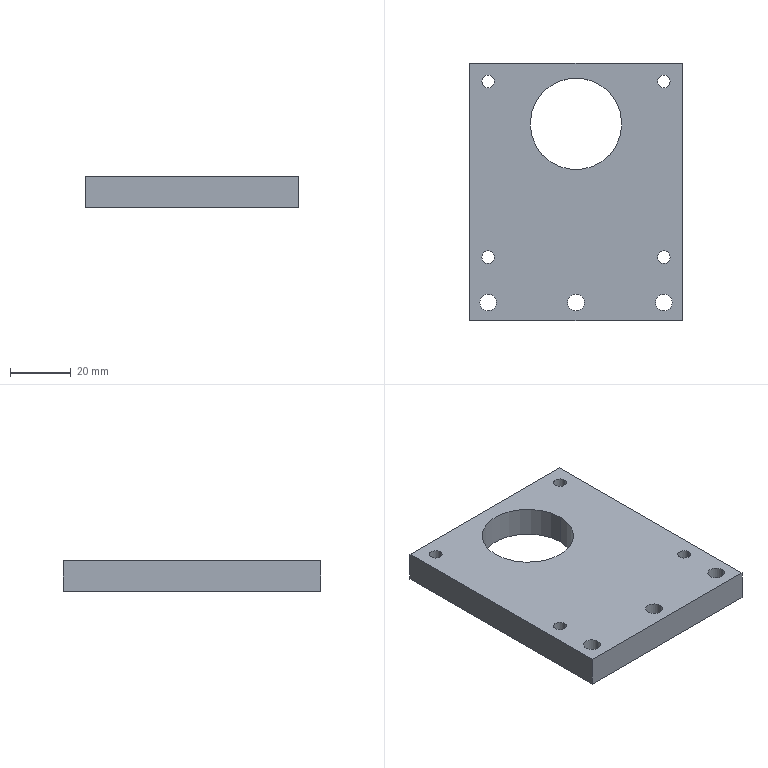Component | SolidWorks | LD101-02--Q1000-Q16-1.SLDQ1SM-1_LD101-02--Q1108-1-1 | 1 solid | 31 faces | box 70 x 85 x 10 mm | volume 50388 mm3 | cylinder 22 | plane 9 | commonest cylinder face diameters 4.2 x8 9 x6 5.5 x6 30.2 x2 | material AL6061
build123d program:
from build123d import *

# Parameters (mm, degrees)
SKETCH1_W                                          = 70
SKETCH1_H                                          = 85
SKETCH1_R                                          = 15.1
BOSS_EXTRUDE1_DEPTH                                = 5
HOLE_SIZE_FOR_HEX_SOCKET_HEAD_CAP_SCRE_D           = 5.5
HOLE_SIZE_FOR_HEX_SOCKET_HEAD_CAP_SCRE_CBORE_D     = 9
HOLE_SIZE_FOR_HEX_SOCKET_HEAD_CAP_SCRE_CBORE_DEPTH = 5.7
M5_TAPPED_HOLE1_D                                  = 4.2


with BuildPart() as part:
    # Sketch1 → Boss-Extrude1 (new, symmetric)
    with BuildSketch(Plane.XY):
        Rectangle(SKETCH1_W, SKETCH1_H)
        with Locations((0, 22.5)):
            Circle(SKETCH1_R, mode=Mode.SUBTRACT)
    extrude(amount=BOSS_EXTRUDE1_DEPTH, both=True)

    # Hole Size _for_ Hex Socket Head Cap Scre (through all)
    with Locations(Plane.XY.offset(5)):
        with Locations((-29, -36.5), (0, -36.5), (29, -36.5)):
            CounterBoreHole(HOLE_SIZE_FOR_HEX_SOCKET_HEAD_CAP_SCRE_D / 2, HOLE_SIZE_FOR_HEX_SOCKET_HEAD_CAP_SCRE_CBORE_D / 2, HOLE_SIZE_FOR_HEX_SOCKET_HEAD_CAP_SCRE_CBORE_DEPTH)

    # M5 Tapped Hole1 (through all)
    with Locations(Plane(origin=(0, 0, -5), x_dir=(-1, 0, 0), z_dir=(0, 0, -1))):
        with Locations((-28.991, -21.491), (28.991, -21.491), (-28.991, 36.491), (28.991, 36.491)):
            Hole(M5_TAPPED_HOLE1_D / 2)


solid = part.part

# Placed as in the assembly
solid = solid.moved(Location((-753.29, -98.397, -75.743), (-180, 0, 180)))
STEP:
#1=CARTESIAN_POINT('',(-30.881,-4.72,-3.179));
#2=VERTEX_POINT('',#1);
#3=CARTESIAN_POINT('',(-30.716,-4.72,-3.179));
#4=VERTEX_POINT('',#3);
#5=CARTESIAN_POINT('',(-30.798,-4.72,-3.179));
#6=DIRECTION('',(-0.,-0.,1.));
#7=DIRECTION('',(1.,0.,0.));
#8=AXIS2_PLACEMENT_3D('',#5,#6,#7);
#9=CIRCLE('',#8,0.08268);
#10=EDGE_CURVE('',#2,#4,#9,.T.);
#11=ORIENTED_EDGE('',*,*,#10,.F.);
#12=CARTESIAN_POINT('',(-30.881,-4.72,-2.785));
#13=VERTEX_POINT('',#12);
#14=CARTESIAN_POINT('',(-30.881,-4.72,-2.785));
#15=DIRECTION('',(-0.,-0.,1.));
#16=VECTOR('',#15,39.37);
#17=LINE('',#14,#16);
#18=EDGE_CURVE('',#2,#13,#17,.T.);
#19=ORIENTED_EDGE('',*,*,#18,.T.);
#20=CARTESIAN_POINT('',(-30.716,-4.72,-2.785));
#21=VERTEX_POINT('',#20);
#22=CARTESIAN_POINT('',(-30.798,-4.72,-2.785));
#23=DIRECTION('',(-0.,-0.,1.));
#24=DIRECTION('',(1.,0.,0.));
#25=AXIS2_PLACEMENT_3D('',#22,#23,#24);
#26=CIRCLE('',#25,0.08268);
#27=EDGE_CURVE('',#13,#21,#26,.T.);
#28=ORIENTED_EDGE('',*,*,#27,.T.);
#29=CARTESIAN_POINT('',(-30.716,-4.72,-2.785));
#30=DIRECTION('',(-0.,-0.,1.));
#31=VECTOR('',#30,39.37);
#32=LINE('',#29,#31);
#33=EDGE_CURVE('',#4,#21,#32,.T.);
#34=ORIENTED_EDGE('',*,*,#33,.F.);
#35=EDGE_LOOP('',(#11,#19,#28,#34));
#36=FACE_OUTER_BOUND('',#35,.T.);
#37=CARTESIAN_POINT('',(-30.798,-4.72,-2.785));
#38=DIRECTION('',(-0.,-0.,1.));
#39=DIRECTION('',(1.,0.,0.));
#40=AXIS2_PLACEMENT_3D('',#37,#38,#39);
#41=CYLINDRICAL_SURFACE('',#40,0.08268);
#42=ADVANCED_FACE('',(#36),#41,.F.);
#43=CARTESIAN_POINT('',(-28.598,-4.72,-3.179));
#44=VERTEX_POINT('',#43);
#45=CARTESIAN_POINT('',(-28.433,-4.72,-3.179));
#46=VERTEX_POINT('',#45);
#47=CARTESIAN_POINT('',(-28.516,-4.72,-3.179));
#48=DIRECTION('',(-0.,-0.,1.));
#49=DIRECTION('',(1.,0.,0.));
#50=AXIS2_PLACEMENT_3D('',#47,#48,#49);
#51=CIRCLE('',#50,0.08268);
#52=EDGE_CURVE('',#44,#46,#51,.T.);
#53=ORIENTED_EDGE('',*,*,#52,.F.);
#54=CARTESIAN_POINT('',(-28.598,-4.72,-2.785));
#55=VERTEX_POINT('',#54);
#56=CARTESIAN_POINT('',(-28.598,-4.72,-2.785));
#57=DIRECTION('',(-0.,-0.,1.));
#58=VECTOR('',#57,39.37);
#59=LINE('',#56,#58);
#60=EDGE_CURVE('',#44,#55,#59,.T.);
#61=ORIENTED_EDGE('',*,*,#60,.T.);
#62=CARTESIAN_POINT('',(-28.433,-4.72,-2.785));
#63=VERTEX_POINT('',#62);
#64=CARTESIAN_POINT('',(-28.516,-4.72,-2.785));
#65=DIRECTION('',(-0.,-0.,1.));
#66=DIRECTION('',(1.,0.,0.));
#67=AXIS2_PLACEMENT_3D('',#64,#65,#66);
#68=CIRCLE('',#67,0.08268);
#69=EDGE_CURVE('',#55,#63,#68,.T.);
#70=ORIENTED_EDGE('',*,*,#69,.T.);
#71=CARTESIAN_POINT('',(-28.433,-4.72,-2.785));
#72=DIRECTION('',(-0.,-0.,1.));
#73=VECTOR('',#72,39.37);
#74=LINE('',#71,#73);
#75=EDGE_CURVE('',#46,#63,#74,.T.);
#76=ORIENTED_EDGE('',*,*,#75,.F.);
#77=EDGE_LOOP('',(#53,#61,#70,#76));
#78=FACE_OUTER_BOUND('',#77,.T.);
#79=CARTESIAN_POINT('',(-28.516,-4.72,-2.785));
#80=DIRECTION('',(-0.,-0.,1.));
#81=DIRECTION('',(1.,0.,0.));
#82=AXIS2_PLACEMENT_3D('',#79,#80,#81);
#83=CYLINDRICAL_SURFACE('',#82,0.08268);
#84=ADVANCED_FACE('',(#78),#83,.F.);
#85=CARTESIAN_POINT('',(-30.881,-2.437,-3.179));
#86=VERTEX_POINT('',#85);
#87=CARTESIAN_POINT('',(-30.716,-2.437,-3.179));
#88=VERTEX_POINT('',#87);
#89=CARTESIAN_POINT('',(-30.798,-2.437,-3.179));
#90=DIRECTION('',(-0.,-0.,1.));
#91=DIRECTION('',(1.,0.,0.));
#92=AXIS2_PLACEMENT_3D('',#89,#90,#91);
#93=CIRCLE('',#92,0.08268);
#94=EDGE_CURVE('',#86,#88,#93,.T.);
#95=ORIENTED_EDGE('',*,*,#94,.F.);
#96=CARTESIAN_POINT('',(-30.881,-2.437,-2.785));
#97=VERTEX_POINT('',#96);
#98=CARTESIAN_POINT('',(-30.881,-2.437,-2.785));
#99=DIRECTION('',(-0.,-0.,1.));
#100=VECTOR('',#99,39.37);
#101=LINE('',#98,#100);
#102=EDGE_CURVE('',#86,#97,#101,.T.);
#103=ORIENTED_EDGE('',*,*,#102,.T.);
#104=CARTESIAN_POINT('',(-30.716,-2.437,-2.785));
#105=VERTEX_POINT('',#104);
#106=CARTESIAN_POINT('',(-30.798,-2.437,-2.785));
#107=DIRECTION('',(-0.,-0.,1.));
#108=DIRECTION('',(1.,0.,0.));
#109=AXIS2_PLACEMENT_3D('',#106,#107,#108);
#110=CIRCLE('',#109,0.08268);
#111=EDGE_CURVE('',#97,#105,#110,.T.);
#112=ORIENTED_EDGE('',*,*,#111,.T.);
#113=CARTESIAN_POINT('',(-30.716,-2.437,-2.785));
#114=DIRECTION('',(-0.,-0.,1.));
#115=VECTOR('',#114,39.37);
#116=LINE('',#113,#115);
#117=EDGE_CURVE('',#88,#105,#116,.T.);
#118=ORIENTED_EDGE('',*,*,#117,.F.);
#119=EDGE_LOOP('',(#95,#103,#112,#118));
#120=FACE_OUTER_BOUND('',#119,.T.);
#121=CARTESIAN_POINT('',(-30.798,-2.437,-2.785));
#122=DIRECTION('',(-0.,-0.,1.));
#123=DIRECTION('',(1.,0.,0.));
#124=AXIS2_PLACEMENT_3D('',#121,#122,#123);
#125=CYLINDRICAL_SURFACE('',#124,0.08268);
#126=ADVANCED_FACE('',(#120),#125,.F.);
#127=CARTESIAN_POINT('',(-28.598,-2.437,-3.179));
#128=VERTEX_POINT('',#127);
#129=CARTESIAN_POINT('',(-28.433,-2.437,-3.179));
#130=VERTEX_POINT('',#129);
#131=CARTESIAN_POINT('',(-28.516,-2.437,-3.179));
#132=DIRECTION('',(-0.,-0.,1.));
#133=DIRECTION('',(1.,0.,0.));
#134=AXIS2_PLACEMENT_3D('',#131,#132,#133);
#135=CIRCLE('',#134,0.08268);
#136=EDGE_CURVE('',#128,#130,#135,.T.);
#137=ORIENTED_EDGE('',*,*,#136,.F.);
#138=CARTESIAN_POINT('',(-28.598,-2.437,-2.785));
#139=VERTEX_POINT('',#138);
#140=CARTESIAN_POINT('',(-28.598,-2.437,-2.785));
#141=DIRECTION('',(-0.,-0.,1.));
#142=VECTOR('',#141,39.37);
#143=LINE('',#140,#142);
#144=EDGE_CURVE('',#128,#139,#143,.T.);
#145=ORIENTED_EDGE('',*,*,#144,.T.);
#146=CARTESIAN_POINT('',(-28.433,-2.437,-2.785));
#147=VERTEX_POINT('',#146);
#148=CARTESIAN_POINT('',(-28.516,-2.437,-2.785));
#149=DIRECTION('',(-0.,-0.,1.));
#150=DIRECTION('',(1.,0.,0.));
#151=AXIS2_PLACEMENT_3D('',#148,#149,#150);
#152=CIRCLE('',#151,0.08268);
#153=EDGE_CURVE('',#139,#147,#152,.T.);
#154=ORIENTED_EDGE('',*,*,#153,.T.);
#155=CARTESIAN_POINT('',(-28.433,-2.437,-2.785));
#156=DIRECTION('',(-0.,-0.,1.));
#157=VECTOR('',#156,39.37);
#158=LINE('',#155,#157);
#159=EDGE_CURVE('',#130,#147,#158,.T.);
#160=ORIENTED_EDGE('',*,*,#159,.F.);
#161=EDGE_LOOP('',(#137,#145,#154,#160));
#162=FACE_OUTER_BOUND('',#161,.T.);
#163=CARTESIAN_POINT('',(-28.516,-2.437,-2.785));
#164=DIRECTION('',(-0.,-0.,1.));
#165=DIRECTION('',(1.,0.,0.));
#166=AXIS2_PLACEMENT_3D('',#163,#164,#165);
#167=CYLINDRICAL_SURFACE('',#166,0.08268);
#168=ADVANCED_FACE('',(#162),#167,.F.);
#169=CARTESIAN_POINT('',(-28.338,-5.311,-2.954));
#170=VERTEX_POINT('',#169);
#171=CARTESIAN_POINT('',(-28.693,-5.311,-2.954));
#172=VERTEX_POINT('',#171);
#173=CARTESIAN_POINT('',(-28.515,-5.311,-2.954));
#174=DIRECTION('',(0.,0.,-1.));
#175=DIRECTION('',(-1.,0.,0.));
#176=AXIS2_PLACEMENT_3D('',#173,#174,#175);
#177=CIRCLE('',#176,0.1772);
#178=EDGE_CURVE('',#170,#172,#177,.T.);
#179=ORIENTED_EDGE('',*,*,#178,.F.);
#180=CARTESIAN_POINT('',(-28.338,-5.311,-3.179));
#181=VERTEX_POINT('',#180);
#182=CARTESIAN_POINT('',(-28.338,-5.311,-3.179));
#183=DIRECTION('',(0.,0.,-1.));
#184=VECTOR('',#183,39.37);
#185=LINE('',#182,#184);
#186=EDGE_CURVE('',#170,#181,#185,.T.);
#187=ORIENTED_EDGE('',*,*,#186,.T.);
#188=CARTESIAN_POINT('',(-28.693,-5.311,-3.179));
#189=VERTEX_POINT('',#188);
#190=CARTESIAN_POINT('',(-28.515,-5.311,-3.179));
#191=DIRECTION('',(0.,0.,-1.));
#192=DIRECTION('',(-1.,0.,0.));
#193=AXIS2_PLACEMENT_3D('',#190,#191,#192);
#194=CIRCLE('',#193,0.1772);
#195=EDGE_CURVE('',#181,#189,#194,.T.);
#196=ORIENTED_EDGE('',*,*,#195,.T.);
#197=CARTESIAN_POINT('',(-28.693,-5.311,-3.179));
#198=DIRECTION('',(0.,0.,-1.));
#199=VECTOR('',#198,39.37);
#200=LINE('',#197,#199);
#201=EDGE_CURVE('',#172,#189,#200,.T.);
#202=ORIENTED_EDGE('',*,*,#201,.F.);
#203=EDGE_LOOP('',(#179,#187,#196,#202));
#204=FACE_OUTER_BOUND('',#203,.T.);
#205=CARTESIAN_POINT('',(-28.515,-5.311,-3.179));
#206=DIRECTION('',(0.,0.,-1.));
#207=DIRECTION('',(-1.,0.,0.));
#208=AXIS2_PLACEMENT_3D('',#205,#206,#207);
#209=CYLINDRICAL_SURFACE('',#208,0.1772);
#210=ADVANCED_FACE('',(#204),#209,.F.);
#211=CARTESIAN_POINT('',(-28.407,-5.311,-2.785));
#212=VERTEX_POINT('',#211);
#213=CARTESIAN_POINT('',(-28.624,-5.311,-2.785));
#214=VERTEX_POINT('',#213);
#215=CARTESIAN_POINT('',(-28.515,-5.311,-2.785));
#216=DIRECTION('',(0.,0.,-1.));
#217=DIRECTION('',(-1.,0.,0.));
#218=AXIS2_PLACEMENT_3D('',#215,#216,#217);
#219=CIRCLE('',#218,0.1083);
#220=EDGE_CURVE('',#212,#214,#219,.T.);
#221=ORIENTED_EDGE('',*,*,#220,.F.);
#222=CARTESIAN_POINT('',(-28.407,-5.311,-2.954));
#223=VERTEX_POINT('',#222);
#224=CARTESIAN_POINT('',(-28.407,-5.311,-3.179));
#225=DIRECTION('',(0.,0.,-1.));
#226=VECTOR('',#225,39.37);
#227=LINE('',#224,#226);
#228=EDGE_CURVE('',#212,#223,#227,.T.);
#229=ORIENTED_EDGE('',*,*,#228,.T.);
#230=CARTESIAN_POINT('',(-28.624,-5.311,-2.954));
#231=VERTEX_POINT('',#230);
#232=CARTESIAN_POINT('',(-28.515,-5.311,-2.954));
#233=DIRECTION('',(0.,0.,-1.));
#234=DIRECTION('',(-1.,0.,0.));
#235=AXIS2_PLACEMENT_3D('',#232,#233,#234);
#236=CIRCLE('',#235,0.1083);
#237=EDGE_CURVE('',#223,#231,#236,.T.);
#238=ORIENTED_EDGE('',*,*,#237,.T.);
#239=CARTESIAN_POINT('',(-28.624,-5.311,-3.179));
#240=DIRECTION('',(0.,0.,-1.));
#241=VECTOR('',#240,39.37);
#242=LINE('',#239,#241);
#243=EDGE_CURVE('',#214,#231,#242,.T.);
#244=ORIENTED_EDGE('',*,*,#243,.F.);
#245=EDGE_LOOP('',(#221,#229,#238,#244));
#246=FACE_OUTER_BOUND('',#245,.T.);
#247=CARTESIAN_POINT('',(-28.515,-5.311,-3.179));
#248=DIRECTION('',(0.,0.,-1.));
#249=DIRECTION('',(-1.,0.,0.));
#250=AXIS2_PLACEMENT_3D('',#247,#248,#249);
#251=CYLINDRICAL_SURFACE('',#250,0.1083);
#252=ADVANCED_FACE('',(#246),#251,.F.);
#253=CARTESIAN_POINT('',(-29.48,-5.311,-2.954));
#254=VERTEX_POINT('',#253);
#255=CARTESIAN_POINT('',(-29.834,-5.311,-2.954));
#256=VERTEX_POINT('',#255);
#257=CARTESIAN_POINT('',(-29.657,-5.311,-2.954));
#258=DIRECTION('',(0.,0.,-1.));
#259=DIRECTION('',(-1.,0.,0.));
#260=AXIS2_PLACEMENT_3D('',#257,#258,#259);
#261=CIRCLE('',#260,0.1772);
#262=EDGE_CURVE('',#254,#256,#261,.T.);
#263=ORIENTED_EDGE('',*,*,#262,.F.);
#264=CARTESIAN_POINT('',(-29.48,-5.311,-3.179));
#265=VERTEX_POINT('',#264);
#266=CARTESIAN_POINT('',(-29.48,-5.311,-3.179));
#267=DIRECTION('',(0.,0.,-1.));
#268=VECTOR('',#267,39.37);
#269=LINE('',#266,#268);
#270=EDGE_CURVE('',#254,#265,#269,.T.);
#271=ORIENTED_EDGE('',*,*,#270,.T.);
#272=CARTESIAN_POINT('',(-29.834,-5.311,-3.179));
#273=VERTEX_POINT('',#272);
#274=CARTESIAN_POINT('',(-29.657,-5.311,-3.179));
#275=DIRECTION('',(0.,0.,-1.));
#276=DIRECTION('',(-1.,0.,0.));
#277=AXIS2_PLACEMENT_3D('',#274,#275,#276);
#278=CIRCLE('',#277,0.1772);
#279=EDGE_CURVE('',#265,#273,#278,.T.);
#280=ORIENTED_EDGE('',*,*,#279,.T.);
#281=CARTESIAN_POINT('',(-29.834,-5.311,-3.179));
#282=DIRECTION('',(0.,0.,-1.));
#283=VECTOR('',#282,39.37);
#284=LINE('',#281,#283);
#285=EDGE_CURVE('',#256,#273,#284,.T.);
#286=ORIENTED_EDGE('',*,*,#285,.F.);
#287=EDGE_LOOP('',(#263,#271,#280,#286));
#288=FACE_OUTER_BOUND('',#287,.T.);
#289=CARTESIAN_POINT('',(-29.657,-5.311,-3.179));
#290=DIRECTION('',(0.,0.,-1.));
#291=DIRECTION('',(-1.,0.,0.));
#292=AXIS2_PLACEMENT_3D('',#289,#290,#291);
#293=CYLINDRICAL_SURFACE('',#292,0.1772);
#294=ADVANCED_FACE('',(#288),#293,.F.);
#295=CARTESIAN_POINT('',(-29.549,-5.311,-2.785));
#296=VERTEX_POINT('',#295);
#297=CARTESIAN_POINT('',(-29.765,-5.311,-2.785));
#298=VERTEX_POINT('',#297);
#299=CARTESIAN_POINT('',(-29.657,-5.311,-2.785));
#300=DIRECTION('',(0.,0.,-1.));
#301=DIRECTION('',(-1.,0.,0.));
#302=AXIS2_PLACEMENT_3D('',#299,#300,#301);
#303=CIRCLE('',#302,0.1083);
#304=EDGE_CURVE('',#296,#298,#303,.T.);
#305=ORIENTED_EDGE('',*,*,#304,.F.);
#306=CARTESIAN_POINT('',(-29.549,-5.311,-2.954));
#307=VERTEX_POINT('',#306);
#308=CARTESIAN_POINT('',(-29.549,-5.311,-3.179));
#309=DIRECTION('',(0.,0.,-1.));
#310=VECTOR('',#309,39.37);
#311=LINE('',#308,#310);
#312=EDGE_CURVE('',#296,#307,#311,.T.);
#313=ORIENTED_EDGE('',*,*,#312,.T.);
#314=CARTESIAN_POINT('',(-29.765,-5.311,-2.954));
#315=VERTEX_POINT('',#314);
#316=CARTESIAN_POINT('',(-29.657,-5.311,-2.954));
#317=DIRECTION('',(0.,0.,-1.));
#318=DIRECTION('',(-1.,0.,0.));
#319=AXIS2_PLACEMENT_3D('',#316,#317,#318);
#320=CIRCLE('',#319,0.1083);
#321=EDGE_CURVE('',#307,#315,#320,.T.);
#322=ORIENTED_EDGE('',*,*,#321,.T.);
#323=CARTESIAN_POINT('',(-29.765,-5.311,-3.179));
#324=DIRECTION('',(0.,0.,-1.));
#325=VECTOR('',#324,39.37);
#326=LINE('',#323,#325);
#327=EDGE_CURVE('',#298,#315,#326,.T.);
#328=ORIENTED_EDGE('',*,*,#327,.F.);
#329=EDGE_LOOP('',(#305,#313,#322,#328));
#330=FACE_OUTER_BOUND('',#329,.T.);
#331=CARTESIAN_POINT('',(-29.657,-5.311,-3.179));
#332=DIRECTION('',(0.,0.,-1.));
#333=DIRECTION('',(-1.,0.,0.));
#334=AXIS2_PLACEMENT_3D('',#331,#332,#333);
#335=CYLINDRICAL_SURFACE('',#334,0.1083);
#336=ADVANCED_FACE('',(#330),#335,.F.);
#337=CARTESIAN_POINT('',(-30.622,-5.311,-2.954));
#338=VERTEX_POINT('',#337);
#339=CARTESIAN_POINT('',(-30.976,-5.311,-2.954));
#340=VERTEX_POINT('',#339);
#341=CARTESIAN_POINT('',(-30.799,-5.311,-2.954));
#342=DIRECTION('',(0.,0.,-1.));
#343=DIRECTION('',(-1.,0.,0.));
#344=AXIS2_PLACEMENT_3D('',#341,#342,#343);
#345=CIRCLE('',#344,0.1772);
#346=EDGE_CURVE('',#338,#340,#345,.T.);
#347=ORIENTED_EDGE('',*,*,#346,.F.);
#348=CARTESIAN_POINT('',(-30.622,-5.311,-3.179));
#349=VERTEX_POINT('',#348);
#350=CARTESIAN_POINT('',(-30.622,-5.311,-3.179));
#351=DIRECTION('',(0.,0.,-1.));
#352=VECTOR('',#351,39.37);
#353=LINE('',#350,#352);
#354=EDGE_CURVE('',#338,#349,#353,.T.);
#355=ORIENTED_EDGE('',*,*,#354,.T.);
#356=CARTESIAN_POINT('',(-30.976,-5.311,-3.179));
#357=VERTEX_POINT('',#356);
#358=CARTESIAN_POINT('',(-30.799,-5.311,-3.179));
#359=DIRECTION('',(0.,0.,-1.));
#360=DIRECTION('',(-1.,0.,0.));
#361=AXIS2_PLACEMENT_3D('',#358,#359,#360);
#362=CIRCLE('',#361,0.1772);
#363=EDGE_CURVE('',#349,#357,#362,.T.);
#364=ORIENTED_EDGE('',*,*,#363,.T.);
#365=CARTESIAN_POINT('',(-30.976,-5.311,-3.179));
#366=DIRECTION('',(0.,0.,-1.));
#367=VECTOR('',#366,39.37);
#368=LINE('',#365,#367);
#369=EDGE_CURVE('',#340,#357,#368,.T.);
#370=ORIENTED_EDGE('',*,*,#369,.F.);
#371=EDGE_LOOP('',(#347,#355,#364,#370));
#372=FACE_OUTER_BOUND('',#371,.T.);
#373=CARTESIAN_POINT('',(-30.799,-5.311,-3.179));
#374=DIRECTION('',(0.,0.,-1.));
#375=DIRECTION('',(-1.,0.,0.));
#376=AXIS2_PLACEMENT_3D('',#373,#374,#375);
#377=CYLINDRICAL_SURFACE('',#376,0.1772);
#378=ADVANCED_FACE('',(#372),#377,.F.);
#379=CARTESIAN_POINT('',(-30.691,-5.311,-2.785));
#380=VERTEX_POINT('',#379);
#381=CARTESIAN_POINT('',(-30.907,-5.311,-2.785));
#382=VERTEX_POINT('',#381);
#383=CARTESIAN_POINT('',(-30.799,-5.311,-2.785));
#384=DIRECTION('',(0.,0.,-1.));
#385=DIRECTION('',(-1.,0.,0.));
#386=AXIS2_PLACEMENT_3D('',#383,#384,#385);
#387=CIRCLE('',#386,0.1083);
#388=EDGE_CURVE('',#380,#382,#387,.T.);
#389=ORIENTED_EDGE('',*,*,#388,.F.);
#390=CARTESIAN_POINT('',(-30.691,-5.311,-2.954));
#391=VERTEX_POINT('',#390);
#392=CARTESIAN_POINT('',(-30.691,-5.311,-3.179));
#393=DIRECTION('',(0.,0.,-1.));
#394=VECTOR('',#393,39.37);
#395=LINE('',#392,#394);
#396=EDGE_CURVE('',#380,#391,#395,.T.);
#397=ORIENTED_EDGE('',*,*,#396,.T.);
#398=CARTESIAN_POINT('',(-30.907,-5.311,-2.954));
#399=VERTEX_POINT('',#398);
#400=CARTESIAN_POINT('',(-30.799,-5.311,-2.954));
#401=DIRECTION('',(0.,0.,-1.));
#402=DIRECTION('',(-1.,0.,0.));
#403=AXIS2_PLACEMENT_3D('',#400,#401,#402);
#404=CIRCLE('',#403,0.1083);
#405=EDGE_CURVE('',#391,#399,#404,.T.);
#406=ORIENTED_EDGE('',*,*,#405,.T.);
#407=CARTESIAN_POINT('',(-30.907,-5.311,-3.179));
#408=DIRECTION('',(0.,0.,-1.));
#409=VECTOR('',#408,39.37);
#410=LINE('',#407,#409);
#411=EDGE_CURVE('',#382,#399,#410,.T.);
#412=ORIENTED_EDGE('',*,*,#411,.F.);
#413=EDGE_LOOP('',(#389,#397,#406,#412));
#414=FACE_OUTER_BOUND('',#413,.T.);
#415=CARTESIAN_POINT('',(-30.799,-5.311,-3.179));
#416=DIRECTION('',(0.,0.,-1.));
#417=DIRECTION('',(-1.,0.,0.));
#418=AXIS2_PLACEMENT_3D('',#415,#416,#417);
#419=CYLINDRICAL_SURFACE('',#418,0.1083);
#420=ADVANCED_FACE('',(#414),#419,.F.);
#421=CARTESIAN_POINT('',(-29.063,-2.988,-3.179));
#422=VERTEX_POINT('',#421);
#423=CARTESIAN_POINT('',(-30.252,-2.988,-3.179));
#424=VERTEX_POINT('',#423);
#425=CARTESIAN_POINT('',(-29.657,-2.988,-3.179));
#426=DIRECTION('',(0.,0.,-1.));
#427=DIRECTION('',(-1.,0.,0.));
#428=AXIS2_PLACEMENT_3D('',#425,#426,#427);
#429=CIRCLE('',#428,0.5945);
#430=EDGE_CURVE('',#422,#424,#429,.T.);
#431=ORIENTED_EDGE('',*,*,#430,.T.);
#432=CARTESIAN_POINT('',(-30.252,-2.988,-2.785));
#433=VERTEX_POINT('',#432);
#434=CARTESIAN_POINT('',(-30.252,-2.988,-3.179));
#435=DIRECTION('',(-0.,-0.,1.));
#436=VECTOR('',#435,39.37);
#437=LINE('',#434,#436);
#438=EDGE_CURVE('',#424,#433,#437,.T.);
#439=ORIENTED_EDGE('',*,*,#438,.T.);
#440=CARTESIAN_POINT('',(-29.063,-2.988,-2.785));
#441=VERTEX_POINT('',#440);
#442=CARTESIAN_POINT('',(-29.657,-2.988,-2.785));
#443=DIRECTION('',(0.,0.,-1.));
#444=DIRECTION('',(-1.,0.,0.));
#445=AXIS2_PLACEMENT_3D('',#442,#443,#444);
#446=CIRCLE('',#445,0.5945);
#447=EDGE_CURVE('',#441,#433,#446,.T.);
#448=ORIENTED_EDGE('',*,*,#447,.F.);
#449=CARTESIAN_POINT('',(-29.063,-2.988,-3.179));
#450=DIRECTION('',(-0.,-0.,1.));
#451=VECTOR('',#450,39.37);
#452=LINE('',#449,#451);
#453=EDGE_CURVE('',#422,#441,#452,.T.);
#454=ORIENTED_EDGE('',*,*,#453,.F.);
#455=EDGE_LOOP('',(#431,#439,#448,#454));
#456=FACE_OUTER_BOUND('',#455,.T.);
#457=CARTESIAN_POINT('',(-29.657,-2.988,-3.179));
#458=DIRECTION('',(-0.,-0.,1.));
#459=DIRECTION('',(1.,0.,0.));
#460=AXIS2_PLACEMENT_3D('',#457,#458,#459);
#461=CYLINDRICAL_SURFACE('',#460,0.5945);
#462=ADVANCED_FACE('',(#456),#461,.F.);
#463=CARTESIAN_POINT('',(-30.798,-4.72,-3.179));
#464=DIRECTION('',(-0.,-0.,1.));
#465=DIRECTION('',(1.,0.,0.));
#466=AXIS2_PLACEMENT_3D('',#463,#464,#465);
#467=CIRCLE('',#466,0.08268);
#468=EDGE_CURVE('',#4,#2,#467,.T.);
#469=ORIENTED_EDGE('',*,*,#468,.T.);
#470=ORIENTED_EDGE('',*,*,#10,.T.);
#471=EDGE_LOOP('',(#469,#470));
#472=FACE_BOUND('',#471,.T.);
#473=CARTESIAN_POINT('',(-28.516,-4.72,-3.179));
#474=DIRECTION('',(-0.,-0.,1.));
#475=DIRECTION('',(1.,0.,0.));
#476=AXIS2_PLACEMENT_3D('',#473,#474,#475);
#477=CIRCLE('',#476,0.08268);
#478=EDGE_CURVE('',#46,#44,#477,.T.);
#479=ORIENTED_EDGE('',*,*,#478,.T.);
#480=ORIENTED_EDGE('',*,*,#52,.T.);
#481=EDGE_LOOP('',(#479,#480));
#482=FACE_BOUND('',#481,.T.);
#483=CARTESIAN_POINT('',(-30.798,-2.437,-3.179));
#484=DIRECTION('',(-0.,-0.,1.));
#485=DIRECTION('',(1.,0.,0.));
#486=AXIS2_PLACEMENT_3D('',#483,#484,#485);
#487=CIRCLE('',#486,0.08268);
#488=EDGE_CURVE('',#88,#86,#487,.T.);
#489=ORIENTED_EDGE('',*,*,#488,.T.);
#490=ORIENTED_EDGE('',*,*,#94,.T.);
#491=EDGE_LOOP('',(#489,#490));
#492=FACE_BOUND('',#491,.T.);
#493=CARTESIAN_POINT('',(-28.516,-2.437,-3.179));
#494=DIRECTION('',(-0.,-0.,1.));
#495=DIRECTION('',(1.,0.,0.));
#496=AXIS2_PLACEMENT_3D('',#493,#494,#495);
#497=CIRCLE('',#496,0.08268);
#498=EDGE_CURVE('',#130,#128,#497,.T.);
#499=ORIENTED_EDGE('',*,*,#498,.T.);
#500=ORIENTED_EDGE('',*,*,#136,.T.);
#501=EDGE_LOOP('',(#499,#500));
#502=FACE_BOUND('',#501,.T.);
#503=CARTESIAN_POINT('',(-28.515,-5.311,-3.179));
#504=DIRECTION('',(0.,0.,-1.));
#505=DIRECTION('',(-1.,0.,0.));
#506=AXIS2_PLACEMENT_3D('',#503,#504,#505);
#507=CIRCLE('',#506,0.1772);
#508=EDGE_CURVE('',#189,#181,#507,.T.);
#509=ORIENTED_EDGE('',*,*,#508,.F.);
#510=ORIENTED_EDGE('',*,*,#195,.F.);
#511=EDGE_LOOP('',(#509,#510));
#512=FACE_BOUND('',#511,.T.);
#513=CARTESIAN_POINT('',(-29.657,-5.311,-3.179));
#514=DIRECTION('',(0.,0.,-1.));
#515=DIRECTION('',(-1.,0.,0.));
#516=AXIS2_PLACEMENT_3D('',#513,#514,#515);
#517=CIRCLE('',#516,0.1772);
#518=EDGE_CURVE('',#273,#265,#517,.T.);
#519=ORIENTED_EDGE('',*,*,#518,.F.);
#520=ORIENTED_EDGE('',*,*,#279,.F.);
#521=EDGE_LOOP('',(#519,#520));
#522=FACE_BOUND('',#521,.T.);
#523=CARTESIAN_POINT('',(-30.799,-5.311,-3.179));
#524=DIRECTION('',(0.,0.,-1.));
#525=DIRECTION('',(-1.,0.,0.));
#526=AXIS2_PLACEMENT_3D('',#523,#524,#525);
#527=CIRCLE('',#526,0.1772);
#528=EDGE_CURVE('',#357,#349,#527,.T.);
#529=ORIENTED_EDGE('',*,*,#528,.F.);
#530=ORIENTED_EDGE('',*,*,#363,.F.);
#531=EDGE_LOOP('',(#529,#530));
#532=FACE_BOUND('',#531,.T.);
#533=CARTESIAN_POINT('',(-31.035,-5.547,-3.179));
#534=VERTEX_POINT('',#533);
#535=CARTESIAN_POINT('',(-31.035,-2.201,-3.179));
#536=VERTEX_POINT('',#535);
#537=CARTESIAN_POINT('',(-31.035,-5.547,-3.179));
#538=DIRECTION('',(0.,1.,0.));
#539=VECTOR('',#538,39.37);
#540=LINE('',#537,#539);
#541=EDGE_CURVE('',#534,#536,#540,.T.);
#542=ORIENTED_EDGE('',*,*,#541,.T.);
#543=CARTESIAN_POINT('',(-28.279,-2.201,-3.179));
#544=VERTEX_POINT('',#543);
#545=CARTESIAN_POINT('',(-28.279,-2.201,-3.179));
#546=DIRECTION('',(1.,-0.,0.));
#547=VECTOR('',#546,39.37);
#548=LINE('',#545,#547);
#549=EDGE_CURVE('',#536,#544,#548,.T.);
#550=ORIENTED_EDGE('',*,*,#549,.T.);
#551=CARTESIAN_POINT('',(-28.279,-5.547,-3.179));
#552=VERTEX_POINT('',#551);
#553=CARTESIAN_POINT('',(-28.279,-5.547,-3.179));
#554=DIRECTION('',(-0.,-1.,-0.));
#555=VECTOR('',#554,39.37);
#556=LINE('',#553,#555);
#557=EDGE_CURVE('',#544,#552,#556,.T.);
#558=ORIENTED_EDGE('',*,*,#557,.T.);
#559=CARTESIAN_POINT('',(-28.279,-5.547,-3.179));
#560=DIRECTION('',(-1.,0.,-0.));
#561=VECTOR('',#560,39.37);
#562=LINE('',#559,#561);
#563=EDGE_CURVE('',#552,#534,#562,.T.);
#564=ORIENTED_EDGE('',*,*,#563,.T.);
#565=EDGE_LOOP('',(#542,#550,#558,#564));
#566=FACE_OUTER_BOUND('',#565,.T.);
#567=ORIENTED_EDGE('',*,*,#430,.F.);
#568=CARTESIAN_POINT('',(-29.657,-2.988,-3.179));
#569=DIRECTION('',(0.,0.,-1.));
#570=DIRECTION('',(-1.,0.,0.));
#571=AXIS2_PLACEMENT_3D('',#568,#569,#570);
#572=CIRCLE('',#571,0.5945);
#573=EDGE_CURVE('',#424,#422,#572,.T.);
#574=ORIENTED_EDGE('',*,*,#573,.F.);
#575=EDGE_LOOP('',(#567,#574));
#576=FACE_BOUND('',#575,.T.);
#577=CARTESIAN_POINT('',(-29.657,-3.874,-3.179));
#578=DIRECTION('',(-0.,-0.,1.));
#579=DIRECTION('',(1.,-0.,0.));
#580=AXIS2_PLACEMENT_3D('',#577,#578,#579);
#581=PLANE('',#580);
#582=ADVANCED_FACE('',(#472,#482,#492,#502,#512,#522,#532,#566,#576),#581,.F.);
#583=CARTESIAN_POINT('',(-30.798,-4.72,-2.785));
#584=DIRECTION('',(-0.,-0.,1.));
#585=DIRECTION('',(1.,0.,0.));
#586=AXIS2_PLACEMENT_3D('',#583,#584,#585);
#587=CIRCLE('',#586,0.08268);
#588=EDGE_CURVE('',#21,#13,#587,.T.);
#589=ORIENTED_EDGE('',*,*,#588,.F.);
#590=ORIENTED_EDGE('',*,*,#27,.F.);
#591=EDGE_LOOP('',(#589,#590));
#592=FACE_BOUND('',#591,.T.);
#593=CARTESIAN_POINT('',(-28.516,-4.72,-2.785));
#594=DIRECTION('',(-0.,-0.,1.));
#595=DIRECTION('',(1.,0.,0.));
#596=AXIS2_PLACEMENT_3D('',#593,#594,#595);
#597=CIRCLE('',#596,0.08268);
#598=EDGE_CURVE('',#63,#55,#597,.T.);
#599=ORIENTED_EDGE('',*,*,#598,.F.);
#600=ORIENTED_EDGE('',*,*,#69,.F.);
#601=EDGE_LOOP('',(#599,#600));
#602=FACE_BOUND('',#601,.T.);
#603=CARTESIAN_POINT('',(-30.798,-2.437,-2.785));
#604=DIRECTION('',(-0.,-0.,1.));
#605=DIRECTION('',(1.,0.,0.));
#606=AXIS2_PLACEMENT_3D('',#603,#604,#605);
#607=CIRCLE('',#606,0.08268);
#608=EDGE_CURVE('',#105,#97,#607,.T.);
#609=ORIENTED_EDGE('',*,*,#608,.F.);
#610=ORIENTED_EDGE('',*,*,#111,.F.);
#611=EDGE_LOOP('',(#609,#610));
#612=FACE_BOUND('',#611,.T.);
#613=CARTESIAN_POINT('',(-28.516,-2.437,-2.785));
#614=DIRECTION('',(-0.,-0.,1.));
#615=DIRECTION('',(1.,0.,0.));
#616=AXIS2_PLACEMENT_3D('',#613,#614,#615);
#617=CIRCLE('',#616,0.08268);
#618=EDGE_CURVE('',#147,#139,#617,.T.);
#619=ORIENTED_EDGE('',*,*,#618,.F.);
#620=ORIENTED_EDGE('',*,*,#153,.F.);
#621=EDGE_LOOP('',(#619,#620));
#622=FACE_BOUND('',#621,.T.);
#623=CARTESIAN_POINT('',(-28.515,-5.311,-2.785));
#624=DIRECTION('',(0.,0.,-1.));
#625=DIRECTION('',(-1.,0.,0.));
#626=AXIS2_PLACEMENT_3D('',#623,#624,#625);
#627=CIRCLE('',#626,0.1083);
#628=EDGE_CURVE('',#214,#212,#627,.T.);
#629=ORIENTED_EDGE('',*,*,#628,.T.);
#630=ORIENTED_EDGE('',*,*,#220,.T.);
#631=EDGE_LOOP('',(#629,#630));
#632=FACE_BOUND('',#631,.T.);
#633=CARTESIAN_POINT('',(-29.657,-5.311,-2.785));
#634=DIRECTION('',(0.,0.,-1.));
#635=DIRECTION('',(-1.,0.,0.));
#636=AXIS2_PLACEMENT_3D('',#633,#634,#635);
#637=CIRCLE('',#636,0.1083);
#638=EDGE_CURVE('',#298,#296,#637,.T.);
#639=ORIENTED_EDGE('',*,*,#638,.T.);
#640=ORIENTED_EDGE('',*,*,#304,.T.);
#641=EDGE_LOOP('',(#639,#640));
#642=FACE_BOUND('',#641,.T.);
#643=CARTESIAN_POINT('',(-30.799,-5.311,-2.785));
#644=DIRECTION('',(0.,0.,-1.));
#645=DIRECTION('',(-1.,0.,0.));
#646=AXIS2_PLACEMENT_3D('',#643,#644,#645);
#647=CIRCLE('',#646,0.1083);
#648=EDGE_CURVE('',#382,#380,#647,.T.);
#649=ORIENTED_EDGE('',*,*,#648,.T.);
#650=ORIENTED_EDGE('',*,*,#388,.T.);
#651=EDGE_LOOP('',(#649,#650));
#652=FACE_BOUND('',#651,.T.);
#653=CARTESIAN_POINT('',(-31.035,-5.547,-2.785));
#654=VERTEX_POINT('',#653);
#655=CARTESIAN_POINT('',(-31.035,-2.201,-2.785));
#656=VERTEX_POINT('',#655);
#657=CARTESIAN_POINT('',(-31.035,-5.547,-2.785));
#658=DIRECTION('',(0.,1.,0.));
#659=VECTOR('',#658,39.37);
#660=LINE('',#657,#659);
#661=EDGE_CURVE('',#654,#656,#660,.T.);
#662=ORIENTED_EDGE('',*,*,#661,.F.);
#663=CARTESIAN_POINT('',(-28.279,-5.547,-2.785));
#664=VERTEX_POINT('',#663);
#665=CARTESIAN_POINT('',(-28.279,-5.547,-2.785));
#666=DIRECTION('',(-1.,0.,-0.));
#667=VECTOR('',#666,39.37);
#668=LINE('',#665,#667);
#669=EDGE_CURVE('',#664,#654,#668,.T.);
#670=ORIENTED_EDGE('',*,*,#669,.F.);
#671=CARTESIAN_POINT('',(-28.279,-2.201,-2.785));
#672=VERTEX_POINT('',#671);
#673=CARTESIAN_POINT('',(-28.279,-5.547,-2.785));
#674=DIRECTION('',(-0.,-1.,-0.));
#675=VECTOR('',#674,39.37);
#676=LINE('',#673,#675);
#677=EDGE_CURVE('',#672,#664,#676,.T.);
#678=ORIENTED_EDGE('',*,*,#677,.F.);
#679=CARTESIAN_POINT('',(-28.279,-2.201,-2.785));
#680=DIRECTION('',(1.,-0.,0.));
#681=VECTOR('',#680,39.37);
#682=LINE('',#679,#681);
#683=EDGE_CURVE('',#656,#672,#682,.T.);
#684=ORIENTED_EDGE('',*,*,#683,.F.);
#685=EDGE_LOOP('',(#662,#670,#678,#684));
#686=FACE_OUTER_BOUND('',#685,.T.);
#687=ORIENTED_EDGE('',*,*,#447,.T.);
#688=CARTESIAN_POINT('',(-29.657,-2.988,-2.785));
#689=DIRECTION('',(0.,0.,-1.));
#690=DIRECTION('',(-1.,0.,0.));
#691=AXIS2_PLACEMENT_3D('',#688,#689,#690);
#692=CIRCLE('',#691,0.5945);
#693=EDGE_CURVE('',#433,#441,#692,.T.);
#694=ORIENTED_EDGE('',*,*,#693,.T.);
#695=EDGE_LOOP('',(#687,#694));
#696=FACE_BOUND('',#695,.T.);
#697=CARTESIAN_POINT('',(-29.657,-3.874,-2.785));
#698=DIRECTION('',(-0.,-0.,1.));
#699=DIRECTION('',(1.,-0.,0.));
#700=AXIS2_PLACEMENT_3D('',#697,#698,#699);
#701=PLANE('',#700);
#702=ADVANCED_FACE('',(#592,#602,#612,#622,#632,#642,#652,#686,#696),#701,.T.);
#703=ORIENTED_EDGE('',*,*,#661,.T.);
#704=CARTESIAN_POINT('',(-31.035,-2.201,-3.179));
#705=DIRECTION('',(-0.,-0.,1.));
#706=VECTOR('',#705,39.37);
#707=LINE('',#704,#706);
#708=EDGE_CURVE('',#536,#656,#707,.T.);
#709=ORIENTED_EDGE('',*,*,#708,.F.);
#710=ORIENTED_EDGE('',*,*,#541,.F.);
#711=CARTESIAN_POINT('',(-31.035,-5.547,-3.179));
#712=DIRECTION('',(-0.,-0.,1.));
#713=VECTOR('',#712,39.37);
#714=LINE('',#711,#713);
#715=EDGE_CURVE('',#534,#654,#714,.T.);
#716=ORIENTED_EDGE('',*,*,#715,.T.);
#717=EDGE_LOOP('',(#703,#709,#710,#716));
#718=FACE_OUTER_BOUND('',#717,.T.);
#719=CARTESIAN_POINT('',(-31.035,-5.547,-3.179));
#720=DIRECTION('',(1.,-0.,0.));
#721=DIRECTION('',(0.,0.,-1.));
#722=AXIS2_PLACEMENT_3D('',#719,#720,#721);
#723=PLANE('',#722);
#724=ADVANCED_FACE('',(#718),#723,.F.);
#725=ORIENTED_EDGE('',*,*,#683,.T.);
#726=CARTESIAN_POINT('',(-28.279,-2.201,-3.179));
#727=DIRECTION('',(-0.,-0.,1.));
#728=VECTOR('',#727,39.37);
#729=LINE('',#726,#728);
#730=EDGE_CURVE('',#544,#672,#729,.T.);
#731=ORIENTED_EDGE('',*,*,#730,.F.);
#732=ORIENTED_EDGE('',*,*,#549,.F.);
#733=ORIENTED_EDGE('',*,*,#708,.T.);
#734=EDGE_LOOP('',(#725,#731,#732,#733));
#735=FACE_OUTER_BOUND('',#734,.T.);
#736=CARTESIAN_POINT('',(-28.279,-2.201,-3.179));
#737=DIRECTION('',(-0.,-1.,-0.));
#738=DIRECTION('',(-0.,-0.,1.));
#739=AXIS2_PLACEMENT_3D('',#736,#737,#738);
#740=PLANE('',#739);
#741=ADVANCED_FACE('',(#735),#740,.F.);
#742=ORIENTED_EDGE('',*,*,#677,.T.);
#743=CARTESIAN_POINT('',(-28.279,-5.547,-3.179));
#744=DIRECTION('',(-0.,-0.,1.));
#745=VECTOR('',#744,39.37);
#746=LINE('',#743,#745);
#747=EDGE_CURVE('',#552,#664,#746,.T.);
#748=ORIENTED_EDGE('',*,*,#747,.F.);
#749=ORIENTED_EDGE('',*,*,#557,.F.);
#750=ORIENTED_EDGE('',*,*,#730,.T.);
#751=EDGE_LOOP('',(#742,#748,#749,#750));
#752=FACE_OUTER_BOUND('',#751,.T.);
#753=CARTESIAN_POINT('',(-28.279,-5.547,-3.179));
#754=DIRECTION('',(-1.,0.,-0.));
#755=DIRECTION('',(-0.,-0.,1.));
#756=AXIS2_PLACEMENT_3D('',#753,#754,#755);
#757=PLANE('',#756);
#758=ADVANCED_FACE('',(#752),#757,.F.);
#759=ORIENTED_EDGE('',*,*,#669,.T.);
#760=ORIENTED_EDGE('',*,*,#715,.F.);
#761=ORIENTED_EDGE('',*,*,#563,.F.);
#762=ORIENTED_EDGE('',*,*,#747,.T.);
#763=EDGE_LOOP('',(#759,#760,#761,#762));
#764=FACE_OUTER_BOUND('',#763,.T.);
#765=CARTESIAN_POINT('',(-28.279,-5.547,-3.179));
#766=DIRECTION('',(0.,1.,0.));
#767=DIRECTION('',(0.,0.,-1.));
#768=AXIS2_PLACEMENT_3D('',#765,#766,#767);
#769=PLANE('',#768);
#770=ADVANCED_FACE('',(#764),#769,.F.);
#771=ORIENTED_EDGE('',*,*,#438,.F.);
#772=ORIENTED_EDGE('',*,*,#573,.T.);
#773=ORIENTED_EDGE('',*,*,#453,.T.);
#774=ORIENTED_EDGE('',*,*,#693,.F.);
#775=EDGE_LOOP('',(#771,#772,#773,#774));
#776=FACE_OUTER_BOUND('',#775,.T.);
#777=CARTESIAN_POINT('',(-29.657,-2.988,-3.179));
#778=DIRECTION('',(-0.,-0.,1.));
#779=DIRECTION('',(1.,0.,0.));
#780=AXIS2_PLACEMENT_3D('',#777,#778,#779);
#781=CYLINDRICAL_SURFACE('',#780,0.5945);
#782=ADVANCED_FACE('',(#776),#781,.F.);
#783=ORIENTED_EDGE('',*,*,#396,.F.);
#784=ORIENTED_EDGE('',*,*,#648,.F.);
#785=ORIENTED_EDGE('',*,*,#411,.T.);
#786=CARTESIAN_POINT('',(-30.799,-5.311,-2.954));
#787=DIRECTION('',(0.,0.,-1.));
#788=DIRECTION('',(-1.,0.,0.));
#789=AXIS2_PLACEMENT_3D('',#786,#787,#788);
#790=CIRCLE('',#789,0.1083);
#791=EDGE_CURVE('',#399,#391,#790,.T.);
#792=ORIENTED_EDGE('',*,*,#791,.T.);
#793=EDGE_LOOP('',(#783,#784,#785,#792));
#794=FACE_OUTER_BOUND('',#793,.T.);
#795=CARTESIAN_POINT('',(-30.799,-5.311,-3.179));
#796=DIRECTION('',(0.,0.,-1.));
#797=DIRECTION('',(-1.,0.,0.));
#798=AXIS2_PLACEMENT_3D('',#795,#796,#797);
#799=CYLINDRICAL_SURFACE('',#798,0.1083);
#800=ADVANCED_FACE('',(#794),#799,.F.);
#801=ORIENTED_EDGE('',*,*,#791,.F.);
#802=ORIENTED_EDGE('',*,*,#405,.F.);
#803=EDGE_LOOP('',(#801,#802));
#804=FACE_BOUND('',#803,.T.);
#805=CARTESIAN_POINT('',(-30.799,-5.311,-2.954));
#806=DIRECTION('',(0.,0.,-1.));
#807=DIRECTION('',(-1.,0.,0.));
#808=AXIS2_PLACEMENT_3D('',#805,#806,#807);
#809=CIRCLE('',#808,0.1772);
#810=EDGE_CURVE('',#340,#338,#809,.T.);
#811=ORIENTED_EDGE('',*,*,#810,.T.);
#812=ORIENTED_EDGE('',*,*,#346,.T.);
#813=EDGE_LOOP('',(#811,#812));
#814=FACE_OUTER_BOUND('',#813,.T.);
#815=CARTESIAN_POINT('',(-30.907,-5.311,-2.954));
#816=DIRECTION('',(-0.,-0.,1.));
#817=DIRECTION('',(1.,-0.,0.));
#818=AXIS2_PLACEMENT_3D('',#815,#816,#817);
#819=PLANE('',#818);
#820=ADVANCED_FACE('',(#804,#814),#819,.F.);
#821=ORIENTED_EDGE('',*,*,#354,.F.);
#822=ORIENTED_EDGE('',*,*,#810,.F.);
#823=ORIENTED_EDGE('',*,*,#369,.T.);
#824=ORIENTED_EDGE('',*,*,#528,.T.);
#825=EDGE_LOOP('',(#821,#822,#823,#824));
#826=FACE_OUTER_BOUND('',#825,.T.);
#827=CARTESIAN_POINT('',(-30.799,-5.311,-3.179));
#828=DIRECTION('',(0.,0.,-1.));
#829=DIRECTION('',(-1.,0.,0.));
#830=AXIS2_PLACEMENT_3D('',#827,#828,#829);
#831=CYLINDRICAL_SURFACE('',#830,0.1772);
#832=ADVANCED_FACE('',(#826),#831,.F.);
#833=ORIENTED_EDGE('',*,*,#312,.F.);
#834=ORIENTED_EDGE('',*,*,#638,.F.);
#835=ORIENTED_EDGE('',*,*,#327,.T.);
#836=CARTESIAN_POINT('',(-29.657,-5.311,-2.954));
#837=DIRECTION('',(0.,0.,-1.));
#838=DIRECTION('',(-1.,0.,0.));
#839=AXIS2_PLACEMENT_3D('',#836,#837,#838);
#840=CIRCLE('',#839,0.1083);
#841=EDGE_CURVE('',#315,#307,#840,.T.);
#842=ORIENTED_EDGE('',*,*,#841,.T.);
#843=EDGE_LOOP('',(#833,#834,#835,#842));
#844=FACE_OUTER_BOUND('',#843,.T.);
#845=CARTESIAN_POINT('',(-29.657,-5.311,-3.179));
#846=DIRECTION('',(0.,0.,-1.));
#847=DIRECTION('',(-1.,0.,0.));
#848=AXIS2_PLACEMENT_3D('',#845,#846,#847);
#849=CYLINDRICAL_SURFACE('',#848,0.1083);
#850=ADVANCED_FACE('',(#844),#849,.F.);
#851=ORIENTED_EDGE('',*,*,#841,.F.);
#852=ORIENTED_EDGE('',*,*,#321,.F.);
#853=EDGE_LOOP('',(#851,#852));
#854=FACE_BOUND('',#853,.T.);
#855=CARTESIAN_POINT('',(-29.657,-5.311,-2.954));
#856=DIRECTION('',(0.,0.,-1.));
#857=DIRECTION('',(-1.,0.,0.));
#858=AXIS2_PLACEMENT_3D('',#855,#856,#857);
#859=CIRCLE('',#858,0.1772);
#860=EDGE_CURVE('',#256,#254,#859,.T.);
#861=ORIENTED_EDGE('',*,*,#860,.T.);
#862=ORIENTED_EDGE('',*,*,#262,.T.);
#863=EDGE_LOOP('',(#861,#862));
#864=FACE_OUTER_BOUND('',#863,.T.);
#865=CARTESIAN_POINT('',(-29.765,-5.311,-2.954));
#866=DIRECTION('',(-0.,-0.,1.));
#867=DIRECTION('',(1.,-0.,0.));
#868=AXIS2_PLACEMENT_3D('',#865,#866,#867);
#869=PLANE('',#868);
#870=ADVANCED_FACE('',(#854,#864),#869,.F.);
#871=ORIENTED_EDGE('',*,*,#270,.F.);
#872=ORIENTED_EDGE('',*,*,#860,.F.);
#873=ORIENTED_EDGE('',*,*,#285,.T.);
#874=ORIENTED_EDGE('',*,*,#518,.T.);
#875=EDGE_LOOP('',(#871,#872,#873,#874));
#876=FACE_OUTER_BOUND('',#875,.T.);
#877=CARTESIAN_POINT('',(-29.657,-5.311,-3.179));
#878=DIRECTION('',(0.,0.,-1.));
#879=DIRECTION('',(-1.,0.,0.));
#880=AXIS2_PLACEMENT_3D('',#877,#878,#879);
#881=CYLINDRICAL_SURFACE('',#880,0.1772);
#882=ADVANCED_FACE('',(#876),#881,.F.);
#883=ORIENTED_EDGE('',*,*,#228,.F.);
#884=ORIENTED_EDGE('',*,*,#628,.F.);
#885=ORIENTED_EDGE('',*,*,#243,.T.);
#886=CARTESIAN_POINT('',(-28.515,-5.311,-2.954));
#887=DIRECTION('',(0.,0.,-1.));
#888=DIRECTION('',(-1.,0.,0.));
#889=AXIS2_PLACEMENT_3D('',#886,#887,#888);
#890=CIRCLE('',#889,0.1083);
#891=EDGE_CURVE('',#231,#223,#890,.T.);
#892=ORIENTED_EDGE('',*,*,#891,.T.);
#893=EDGE_LOOP('',(#883,#884,#885,#892));
#894=FACE_OUTER_BOUND('',#893,.T.);
#895=CARTESIAN_POINT('',(-28.515,-5.311,-3.179));
#896=DIRECTION('',(0.,0.,-1.));
#897=DIRECTION('',(-1.,0.,0.));
#898=AXIS2_PLACEMENT_3D('',#895,#896,#897);
#899=CYLINDRICAL_SURFACE('',#898,0.1083);
#900=ADVANCED_FACE('',(#894),#899,.F.);
#901=ORIENTED_EDGE('',*,*,#891,.F.);
#902=ORIENTED_EDGE('',*,*,#237,.F.);
#903=EDGE_LOOP('',(#901,#902));
#904=FACE_BOUND('',#903,.T.);
#905=CARTESIAN_POINT('',(-28.515,-5.311,-2.954));
#906=DIRECTION('',(0.,0.,-1.));
#907=DIRECTION('',(-1.,0.,0.));
#908=AXIS2_PLACEMENT_3D('',#905,#906,#907);
#909=CIRCLE('',#908,0.1772);
#910=EDGE_CURVE('',#172,#170,#909,.T.);
#911=ORIENTED_EDGE('',*,*,#910,.T.);
#912=ORIENTED_EDGE('',*,*,#178,.T.);
#913=EDGE_LOOP('',(#911,#912));
#914=FACE_OUTER_BOUND('',#913,.T.);
#915=CARTESIAN_POINT('',(-28.624,-5.311,-2.954));
#916=DIRECTION('',(-0.,-0.,1.));
#917=DIRECTION('',(1.,-0.,0.));
#918=AXIS2_PLACEMENT_3D('',#915,#916,#917);
#919=PLANE('',#918);
#920=ADVANCED_FACE('',(#904,#914),#919,.F.);
#921=ORIENTED_EDGE('',*,*,#186,.F.);
#922=ORIENTED_EDGE('',*,*,#910,.F.);
#923=ORIENTED_EDGE('',*,*,#201,.T.);
#924=ORIENTED_EDGE('',*,*,#508,.T.);
#925=EDGE_LOOP('',(#921,#922,#923,#924));
#926=FACE_OUTER_BOUND('',#925,.T.);
#927=CARTESIAN_POINT('',(-28.515,-5.311,-3.179));
#928=DIRECTION('',(0.,0.,-1.));
#929=DIRECTION('',(-1.,0.,0.));
#930=AXIS2_PLACEMENT_3D('',#927,#928,#929);
#931=CYLINDRICAL_SURFACE('',#930,0.1772);
#932=ADVANCED_FACE('',(#926),#931,.F.);
#933=ORIENTED_EDGE('',*,*,#144,.F.);
#934=ORIENTED_EDGE('',*,*,#498,.F.);
#935=ORIENTED_EDGE('',*,*,#159,.T.);
#936=ORIENTED_EDGE('',*,*,#618,.T.);
#937=EDGE_LOOP('',(#933,#934,#935,#936));
#938=FACE_OUTER_BOUND('',#937,.T.);
#939=CARTESIAN_POINT('',(-28.516,-2.437,-2.785));
#940=DIRECTION('',(-0.,-0.,1.));
#941=DIRECTION('',(1.,0.,0.));
#942=AXIS2_PLACEMENT_3D('',#939,#940,#941);
#943=CYLINDRICAL_SURFACE('',#942,0.08268);
#944=ADVANCED_FACE('',(#938),#943,.F.);
#945=ORIENTED_EDGE('',*,*,#102,.F.);
#946=ORIENTED_EDGE('',*,*,#488,.F.);
#947=ORIENTED_EDGE('',*,*,#117,.T.);
#948=ORIENTED_EDGE('',*,*,#608,.T.);
#949=EDGE_LOOP('',(#945,#946,#947,#948));
#950=FACE_OUTER_BOUND('',#949,.T.);
#951=CARTESIAN_POINT('',(-30.798,-2.437,-2.785));
#952=DIRECTION('',(-0.,-0.,1.));
#953=DIRECTION('',(1.,0.,0.));
#954=AXIS2_PLACEMENT_3D('',#951,#952,#953);
#955=CYLINDRICAL_SURFACE('',#954,0.08268);
#956=ADVANCED_FACE('',(#950),#955,.F.);
#957=ORIENTED_EDGE('',*,*,#60,.F.);
#958=ORIENTED_EDGE('',*,*,#478,.F.);
#959=ORIENTED_EDGE('',*,*,#75,.T.);
#960=ORIENTED_EDGE('',*,*,#598,.T.);
#961=EDGE_LOOP('',(#957,#958,#959,#960));
#962=FACE_OUTER_BOUND('',#961,.T.);
#963=CARTESIAN_POINT('',(-28.516,-4.72,-2.785));
#964=DIRECTION('',(-0.,-0.,1.));
#965=DIRECTION('',(1.,0.,0.));
#966=AXIS2_PLACEMENT_3D('',#963,#964,#965);
#967=CYLINDRICAL_SURFACE('',#966,0.08268);
#968=ADVANCED_FACE('',(#962),#967,.F.);
#969=ORIENTED_EDGE('',*,*,#18,.F.);
#970=ORIENTED_EDGE('',*,*,#468,.F.);
#971=ORIENTED_EDGE('',*,*,#33,.T.);
#972=ORIENTED_EDGE('',*,*,#588,.T.);
#973=EDGE_LOOP('',(#969,#970,#971,#972));
#974=FACE_OUTER_BOUND('',#973,.T.);
#975=CARTESIAN_POINT('',(-30.798,-4.72,-2.785));
#976=DIRECTION('',(-0.,-0.,1.));
#977=DIRECTION('',(1.,0.,0.));
#978=AXIS2_PLACEMENT_3D('',#975,#976,#977);
#979=CYLINDRICAL_SURFACE('',#978,0.08268);
#980=ADVANCED_FACE('',(#974),#979,.F.);
#981=CLOSED_SHELL('',(#42,#84,#126,#168,#210,#252,#294,#336,#378,#420,#462,#582,#702,#724,#741,#758,#770,#782,#800,#820,#832,#850,#870,#882,#900,#920,#932,#944,#956,#968,#980));
#982=MANIFOLD_SOLID_BREP('',#981);
#983=CARTESIAN_POINT('',(0.,0.,0.));
#984=DIRECTION('',(0.,0.,1.));
#985=DIRECTION('',(1.,0.,0.));
#986=AXIS2_PLACEMENT_3D('',#983,#984,#985);
#987=(LENGTH_UNIT()NAMED_UNIT(*)SI_UNIT($,.METRE.));
#988=LENGTH_MEASURE_WITH_UNIT(LENGTH_MEASURE(0.0254),#987);
#989=DIMENSIONAL_EXPONENTS(1.,0.,0.,0.,0.,0.,0.);
#990=(CONVERSION_BASED_UNIT('',#988)LENGTH_UNIT()NAMED_UNIT(#989));
#991=UNCERTAINTY_MEASURE_WITH_UNIT(LENGTH_MEASURE(0.00001),#990,'','');
#992=(NAMED_UNIT(*)PLANE_ANGLE_UNIT()SI_UNIT($,.RADIAN.));
#993=(NAMED_UNIT(*)SI_UNIT($,.STERADIAN.)SOLID_ANGLE_UNIT());
#994=(GEOMETRIC_REPRESENTATION_CONTEXT(3)GLOBAL_UNCERTAINTY_ASSIGNED_CONTEXT((#991))GLOBAL_UNIT_ASSIGNED_CONTEXT((#990,#992,#993))REPRESENTATION_CONTEXT('',''));
#995=ADVANCED_BREP_SHAPE_REPRESENTATION('',(#982,#986),#994);
#996=COLOUR_RGB('',0.7922,0.8196,0.9333);
#997=FILL_AREA_STYLE_COLOUR('',#996);
#998=FILL_AREA_STYLE('',(#997));
#999=SURFACE_STYLE_FILL_AREA(#998);
#1000=SURFACE_SIDE_STYLE('',(#999));
#1001=SURFACE_STYLE_USAGE(.BOTH.,#1000);
#1002=PRESENTATION_STYLE_ASSIGNMENT((#1001));
#1003=STYLED_ITEM('',(#1002),#982);
#1004=PRESENTATION_LAYER_ASSIGNMENT('','',(#1003));
#1005=(LENGTH_UNIT()NAMED_UNIT(*)SI_UNIT($,.METRE.));
#1006=LENGTH_MEASURE_WITH_UNIT(LENGTH_MEASURE(0.0254),#1005);
#1007=DIMENSIONAL_EXPONENTS(1.,0.,0.,0.,0.,0.,0.);
#1008=(CONVERSION_BASED_UNIT('',#1006)LENGTH_UNIT()NAMED_UNIT(#1007));
#1009=UNCERTAINTY_MEASURE_WITH_UNIT(LENGTH_MEASURE(0.00001),#1008,'','');
#1010=(NAMED_UNIT(*)PLANE_ANGLE_UNIT()SI_UNIT($,.RADIAN.));
#1011=(NAMED_UNIT(*)SI_UNIT($,.STERADIAN.)SOLID_ANGLE_UNIT());
#1012=(GEOMETRIC_REPRESENTATION_CONTEXT(3)GLOBAL_UNCERTAINTY_ASSIGNED_CONTEXT((#1009))GLOBAL_UNIT_ASSIGNED_CONTEXT((#1008,#1010,#1011))REPRESENTATION_CONTEXT('',''));
#1013=MECHANICAL_DESIGN_GEOMETRIC_PRESENTATION_REPRESENTATION('',(#1003),#1012);